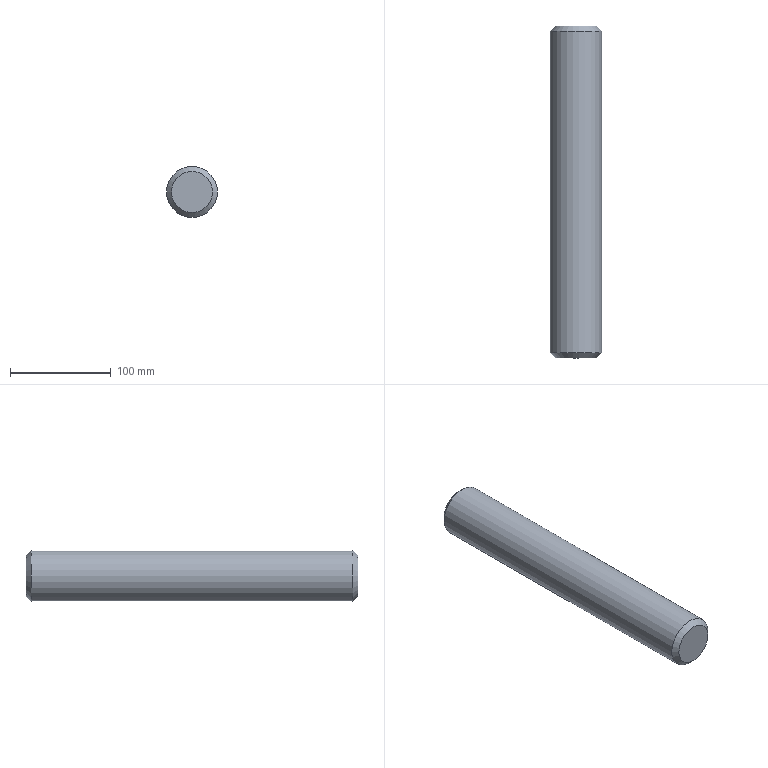Component | NX | PIN_330 | 1 solid | 5 faces | volume 665126 mm3 | plane 2 | cone 2 | cylinder 1 | commonest cylinder face diameters 50.8 x1